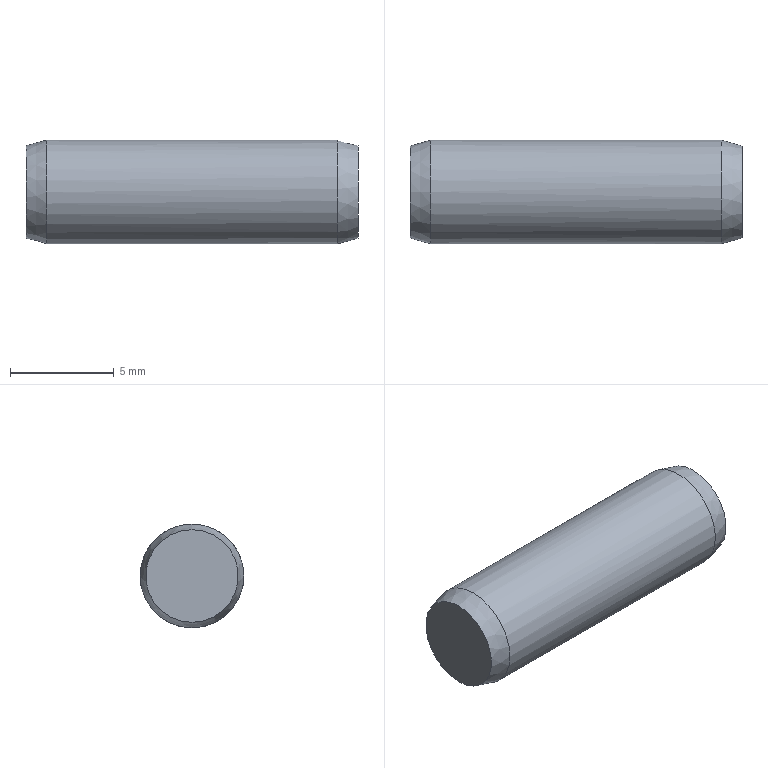Component | NX | PIN | 1 solid | 5 faces | box 16 x 5 x 5 mm | volume 310 mm3 | plane 2 | cone 2 | cylinder 1 | commonest cylinder face diameters 5 x1
STEP:
#1=CARTESIAN_POINT('',(0.,0.,0.));
#2=DIRECTION('',(0.,0.,1.));
#3=DIRECTION('',(1.,0.,0.));
#4=AXIS2_PLACEMENT_3D('',#1,#2,#3);
#5=CARTESIAN_POINT('',(8.5,25.456,32.724));
#6=VERTEX_POINT('',#5);
#7=CARTESIAN_POINT('',(8.5,25.456,34.956));
#8=DIRECTION('',(1.,0.,0.));
#9=DIRECTION('',(0.,0.,-1.));
#10=AXIS2_PLACEMENT_3D('',#7,#8,#9);
#11=CIRCLE('',#10,2.232);
#12=CARTESIAN_POINT('',(8.5,25.456,34.956));
#13=DIRECTION('',(1.,0.,0.));
#14=DIRECTION('',(0.,0.,-1.));
#15=AXIS2_PLACEMENT_3D('',#12,#13,#14);
#16=PLANE('',#15);
#17=CARTESIAN_POINT('',(0.,0.));
#18=DIRECTION('',(1.,0.));
#19=AXIS2_PLACEMENT_2D('',#17,#18);
#20=CIRCLE('',#19,2.232);
#21=(GEOMETRIC_REPRESENTATION_CONTEXT(2)PARAMETRIC_REPRESENTATION_CONTEXT()REPRESENTATION_CONTEXT('',''));
#22=DEFINITIONAL_REPRESENTATION('',(#20),#21);
#23=PCURVE('',#16,#22);
#24=CARTESIAN_POINT('',(7.5,25.456,34.956));
#25=DIRECTION('',(-1.,0.,0.));
#26=DIRECTION('',(0.,0.,1.));
#27=AXIS2_PLACEMENT_3D('',#24,#25,#26);
#28=CONICAL_SURFACE('',#27,2.5,0.2618);
#29=CARTESIAN_POINT('',(9.425,-1.));
#30=DIRECTION('',(-1.,0.));
#31=VECTOR('',#30,1.);
#32=LINE('',#29,#31);
#33=(GEOMETRIC_REPRESENTATION_CONTEXT(2)PARAMETRIC_REPRESENTATION_CONTEXT()REPRESENTATION_CONTEXT('',''));
#34=DEFINITIONAL_REPRESENTATION('',(#32),#33);
#35=PCURVE('',#28,#34);
#36=SURFACE_CURVE('',#11,(#23,#35),.PCURVE_S1.);
#37=EDGE_CURVE('',#6,#6,#36,.T.);
#38=ORIENTED_EDGE('',*,*,#37,.T.);
#39=EDGE_LOOP('',(#38));
#40=FACE_BOUND('',#39,.T.);
#41=ADVANCED_FACE('',(#40),#16,.T.);
#42=CARTESIAN_POINT('',(-7.5,25.456,37.188));
#43=VERTEX_POINT('',#42);
#44=CARTESIAN_POINT('',(-7.5,25.456,34.956));
#45=DIRECTION('',(-1.,0.,0.));
#46=DIRECTION('',(0.,0.,1.));
#47=AXIS2_PLACEMENT_3D('',#44,#45,#46);
#48=CIRCLE('',#47,2.232);
#49=CARTESIAN_POINT('',(-7.5,25.456,34.956));
#50=DIRECTION('',(-1.,0.,0.));
#51=DIRECTION('',(0.,0.,1.));
#52=AXIS2_PLACEMENT_3D('',#49,#50,#51);
#53=PLANE('',#52);
#54=CARTESIAN_POINT('',(0.,0.));
#55=DIRECTION('',(1.,0.));
#56=AXIS2_PLACEMENT_2D('',#54,#55);
#57=CIRCLE('',#56,2.232);
#58=(GEOMETRIC_REPRESENTATION_CONTEXT(2)PARAMETRIC_REPRESENTATION_CONTEXT()REPRESENTATION_CONTEXT('',''));
#59=DEFINITIONAL_REPRESENTATION('',(#57),#58);
#60=PCURVE('',#53,#59);
#61=CARTESIAN_POINT('',(-6.5,25.456,34.956));
#62=DIRECTION('',(1.,0.,0.));
#63=DIRECTION('',(0.,0.,-1.));
#64=AXIS2_PLACEMENT_3D('',#61,#62,#63);
#65=CONICAL_SURFACE('',#64,2.5,0.2618);
#66=CARTESIAN_POINT('',(9.425,-1.));
#67=DIRECTION('',(-1.,0.));
#68=VECTOR('',#67,1.);
#69=LINE('',#66,#68);
#70=(GEOMETRIC_REPRESENTATION_CONTEXT(2)PARAMETRIC_REPRESENTATION_CONTEXT()REPRESENTATION_CONTEXT('',''));
#71=DEFINITIONAL_REPRESENTATION('',(#69),#70);
#72=PCURVE('',#65,#71);
#73=SURFACE_CURVE('',#48,(#60,#72),.PCURVE_S1.);
#74=EDGE_CURVE('',#43,#43,#73,.T.);
#75=ORIENTED_EDGE('',*,*,#74,.T.);
#76=EDGE_LOOP('',(#75));
#77=FACE_BOUND('',#76,.T.);
#78=ADVANCED_FACE('',(#77),#53,.T.);
#79=CARTESIAN_POINT('',(-6.5,25.456,37.456));
#80=VERTEX_POINT('',#79);
#81=CARTESIAN_POINT('',(-6.5,25.456,32.456));
#82=VERTEX_POINT('',#81);
#83=CARTESIAN_POINT('',(-6.5,25.456,34.956));
#84=DIRECTION('',(1.,0.,0.));
#85=DIRECTION('',(0.,0.,1.));
#86=AXIS2_PLACEMENT_3D('',#83,#84,#85);
#87=CIRCLE('',#86,2.5);
#88=CARTESIAN_POINT('',(-7.5,25.456,34.956));
#89=DIRECTION('',(1.,0.,0.));
#90=DIRECTION('',(0.,0.,-1.));
#91=AXIS2_PLACEMENT_3D('',#88,#89,#90);
#92=CYLINDRICAL_SURFACE('',#91,2.5);
#93=CARTESIAN_POINT('',(3.142,1.));
#94=DIRECTION('',(1.,0.));
#95=VECTOR('',#94,1.);
#96=LINE('',#93,#95);
#97=(GEOMETRIC_REPRESENTATION_CONTEXT(2)PARAMETRIC_REPRESENTATION_CONTEXT()REPRESENTATION_CONTEXT('',''));
#98=DEFINITIONAL_REPRESENTATION('',(#96),#97);
#99=PCURVE('',#92,#98);
#100=CARTESIAN_POINT('',(3.142,0.));
#101=DIRECTION('',(1.,0.));
#102=VECTOR('',#101,1.);
#103=LINE('',#100,#102);
#104=(GEOMETRIC_REPRESENTATION_CONTEXT(2)PARAMETRIC_REPRESENTATION_CONTEXT()REPRESENTATION_CONTEXT('',''));
#105=DEFINITIONAL_REPRESENTATION('',(#103),#104);
#106=PCURVE('',#65,#105);
#107=SURFACE_CURVE('',#87,(#99,#106),.PCURVE_S1.);
#108=EDGE_CURVE('',#80,#82,#107,.T.);
#109=ORIENTED_EDGE('',*,*,#108,.T.);
#110=CARTESIAN_POINT('',(7.5,25.456,32.456));
#111=VERTEX_POINT('',#110);
#112=CARTESIAN_POINT('',(-6.5,25.456,32.456));
#113=CARTESIAN_POINT('',(7.5,25.456,32.456));
#114=B_SPLINE_CURVE_WITH_KNOTS('',1,(#112,#113),.UNSPECIFIED.,.F.,.F.,(2,2),(1.,15.),.PIECEWISE_BEZIER_KNOTS.);
#115=CARTESIAN_POINT('',(6.283,0.));
#116=DIRECTION('',(0.,1.));
#117=VECTOR('',#116,1.);
#118=LINE('',#115,#117);
#119=(GEOMETRIC_REPRESENTATION_CONTEXT(2)PARAMETRIC_REPRESENTATION_CONTEXT()REPRESENTATION_CONTEXT('',''));
#120=DEFINITIONAL_REPRESENTATION('',(#118),#119);
#121=PCURVE('',#92,#120);
#122=CARTESIAN_POINT('',(0.,0.));
#123=DIRECTION('',(0.,1.));
#124=VECTOR('',#123,1.);
#125=LINE('',#122,#124);
#126=(GEOMETRIC_REPRESENTATION_CONTEXT(2)PARAMETRIC_REPRESENTATION_CONTEXT()REPRESENTATION_CONTEXT('',''));
#127=DEFINITIONAL_REPRESENTATION('',(#125),#126);
#128=PCURVE('',#92,#127);
#129=SEAM_CURVE('',#114,(#121,#128),.PCURVE_S1.);
#130=EDGE_CURVE('',#82,#111,#129,.T.);
#131=ORIENTED_EDGE('',*,*,#130,.T.);
#132=CARTESIAN_POINT('',(7.5,25.456,34.956));
#133=DIRECTION('',(-1.,0.,0.));
#134=DIRECTION('',(0.,0.,-1.));
#135=AXIS2_PLACEMENT_3D('',#132,#133,#134);
#136=CIRCLE('',#135,2.5);
#137=CARTESIAN_POINT('',(6.283,15.));
#138=DIRECTION('',(-1.,0.));
#139=VECTOR('',#138,1.);
#140=LINE('',#137,#139);
#141=(GEOMETRIC_REPRESENTATION_CONTEXT(2)PARAMETRIC_REPRESENTATION_CONTEXT()REPRESENTATION_CONTEXT('',''));
#142=DEFINITIONAL_REPRESENTATION('',(#140),#141);
#143=PCURVE('',#92,#142);
#144=CARTESIAN_POINT('',(3.142,0.));
#145=DIRECTION('',(1.,0.));
#146=VECTOR('',#145,1.);
#147=LINE('',#144,#146);
#148=(GEOMETRIC_REPRESENTATION_CONTEXT(2)PARAMETRIC_REPRESENTATION_CONTEXT()REPRESENTATION_CONTEXT('',''));
#149=DEFINITIONAL_REPRESENTATION('',(#147),#148);
#150=PCURVE('',#28,#149);
#151=SURFACE_CURVE('',#136,(#143,#150),.PCURVE_S1.);
#152=EDGE_CURVE('',#111,#111,#151,.T.);
#153=ORIENTED_EDGE('',*,*,#152,.T.);
#154=ORIENTED_EDGE('',*,*,#130,.F.);
#155=CARTESIAN_POINT('',(-6.5,25.456,34.956));
#156=DIRECTION('',(1.,0.,0.));
#157=DIRECTION('',(0.,0.,1.));
#158=AXIS2_PLACEMENT_3D('',#155,#156,#157);
#159=CIRCLE('',#158,2.5);
#160=CARTESIAN_POINT('',(-3.142,1.));
#161=DIRECTION('',(1.,0.));
#162=VECTOR('',#161,1.);
#163=LINE('',#160,#162);
#164=(GEOMETRIC_REPRESENTATION_CONTEXT(2)PARAMETRIC_REPRESENTATION_CONTEXT()REPRESENTATION_CONTEXT('',''));
#165=DEFINITIONAL_REPRESENTATION('',(#163),#164);
#166=PCURVE('',#92,#165);
#167=CARTESIAN_POINT('',(3.142,0.));
#168=DIRECTION('',(1.,0.));
#169=VECTOR('',#168,1.);
#170=LINE('',#167,#169);
#171=(GEOMETRIC_REPRESENTATION_CONTEXT(2)PARAMETRIC_REPRESENTATION_CONTEXT()REPRESENTATION_CONTEXT('',''));
#172=DEFINITIONAL_REPRESENTATION('',(#170),#171);
#173=PCURVE('',#65,#172);
#174=SURFACE_CURVE('',#159,(#166,#173),.PCURVE_S1.);
#175=EDGE_CURVE('',#82,#80,#174,.T.);
#176=ORIENTED_EDGE('',*,*,#175,.T.);
#177=EDGE_LOOP('',(#109,#131,#153,#154,#176));
#178=FACE_BOUND('',#177,.T.);
#179=ADVANCED_FACE('',(#178),#92,.T.);
#180=ORIENTED_EDGE('',*,*,#37,.F.);
#181=CARTESIAN_POINT('',(8.5,25.456,32.724));
#182=CARTESIAN_POINT('',(7.5,25.456,32.456));
#183=B_SPLINE_CURVE_WITH_KNOTS('',1,(#181,#182),.UNSPECIFIED.,.F.,.F.,(2,2),(-1.035,0.),.PIECEWISE_BEZIER_KNOTS.);
#184=CARTESIAN_POINT('',(9.425,0.));
#185=DIRECTION('',(0.,1.));
#186=VECTOR('',#185,1.);
#187=LINE('',#184,#186);
#188=(GEOMETRIC_REPRESENTATION_CONTEXT(2)PARAMETRIC_REPRESENTATION_CONTEXT()REPRESENTATION_CONTEXT('',''));
#189=DEFINITIONAL_REPRESENTATION('',(#187),#188);
#190=PCURVE('',#28,#189);
#191=CARTESIAN_POINT('',(3.142,0.));
#192=DIRECTION('',(0.,1.));
#193=VECTOR('',#192,1.);
#194=LINE('',#191,#193);
#195=(GEOMETRIC_REPRESENTATION_CONTEXT(2)PARAMETRIC_REPRESENTATION_CONTEXT()REPRESENTATION_CONTEXT('',''));
#196=DEFINITIONAL_REPRESENTATION('',(#194),#195);
#197=PCURVE('',#28,#196);
#198=SEAM_CURVE('',#183,(#190,#197),.PCURVE_S1.);
#199=EDGE_CURVE('',#6,#111,#198,.T.);
#200=ORIENTED_EDGE('',*,*,#199,.T.);
#201=ORIENTED_EDGE('',*,*,#152,.F.);
#202=ORIENTED_EDGE('',*,*,#199,.F.);
#203=EDGE_LOOP('',(#180,#200,#201,#202));
#204=FACE_BOUND('',#203,.T.);
#205=ADVANCED_FACE('',(#204),#28,.T.);
#206=ORIENTED_EDGE('',*,*,#74,.F.);
#207=CARTESIAN_POINT('',(-7.5,25.456,37.188));
#208=CARTESIAN_POINT('',(-6.5,25.456,37.456));
#209=B_SPLINE_CURVE_WITH_KNOTS('',1,(#207,#208),.UNSPECIFIED.,.F.,.F.,(2,2),(-1.035,0.),.PIECEWISE_BEZIER_KNOTS.);
#210=CARTESIAN_POINT('',(9.425,0.));
#211=DIRECTION('',(0.,1.));
#212=VECTOR('',#211,1.);
#213=LINE('',#210,#212);
#214=(GEOMETRIC_REPRESENTATION_CONTEXT(2)PARAMETRIC_REPRESENTATION_CONTEXT()REPRESENTATION_CONTEXT('',''));
#215=DEFINITIONAL_REPRESENTATION('',(#213),#214);
#216=PCURVE('',#65,#215);
#217=CARTESIAN_POINT('',(3.142,0.));
#218=DIRECTION('',(0.,1.));
#219=VECTOR('',#218,1.);
#220=LINE('',#217,#219);
#221=(GEOMETRIC_REPRESENTATION_CONTEXT(2)PARAMETRIC_REPRESENTATION_CONTEXT()REPRESENTATION_CONTEXT('',''));
#222=DEFINITIONAL_REPRESENTATION('',(#220),#221);
#223=PCURVE('',#65,#222);
#224=SEAM_CURVE('',#209,(#216,#223),.PCURVE_S1.);
#225=EDGE_CURVE('',#43,#80,#224,.T.);
#226=ORIENTED_EDGE('',*,*,#225,.T.);
#227=ORIENTED_EDGE('',*,*,#175,.F.);
#228=ORIENTED_EDGE('',*,*,#108,.F.);
#229=ORIENTED_EDGE('',*,*,#225,.F.);
#230=EDGE_LOOP('',(#206,#226,#227,#228,#229));
#231=FACE_BOUND('',#230,.T.);
#232=ADVANCED_FACE('',(#231),#65,.T.);
#233=CLOSED_SHELL('',(#41,#78,#179,#205,#232));
#234=MANIFOLD_SOLID_BREP('',#233);
#235=(LENGTH_UNIT()NAMED_UNIT(*)SI_UNIT(.MILLI.,.METRE.));
#236=UNCERTAINTY_MEASURE_WITH_UNIT(LENGTH_MEASURE(0.00001),#235,'','');
#237=(NAMED_UNIT(*)PLANE_ANGLE_UNIT()SI_UNIT($,.RADIAN.));
#238=(NAMED_UNIT(*)SI_UNIT($,.STERADIAN.)SOLID_ANGLE_UNIT());
#239=(GEOMETRIC_REPRESENTATION_CONTEXT(3)GLOBAL_UNCERTAINTY_ASSIGNED_CONTEXT((#236))GLOBAL_UNIT_ASSIGNED_CONTEXT((#235,#237,#238))REPRESENTATION_CONTEXT('',''));
#240=ADVANCED_BREP_SHAPE_REPRESENTATION('',(#4,#234),#239);